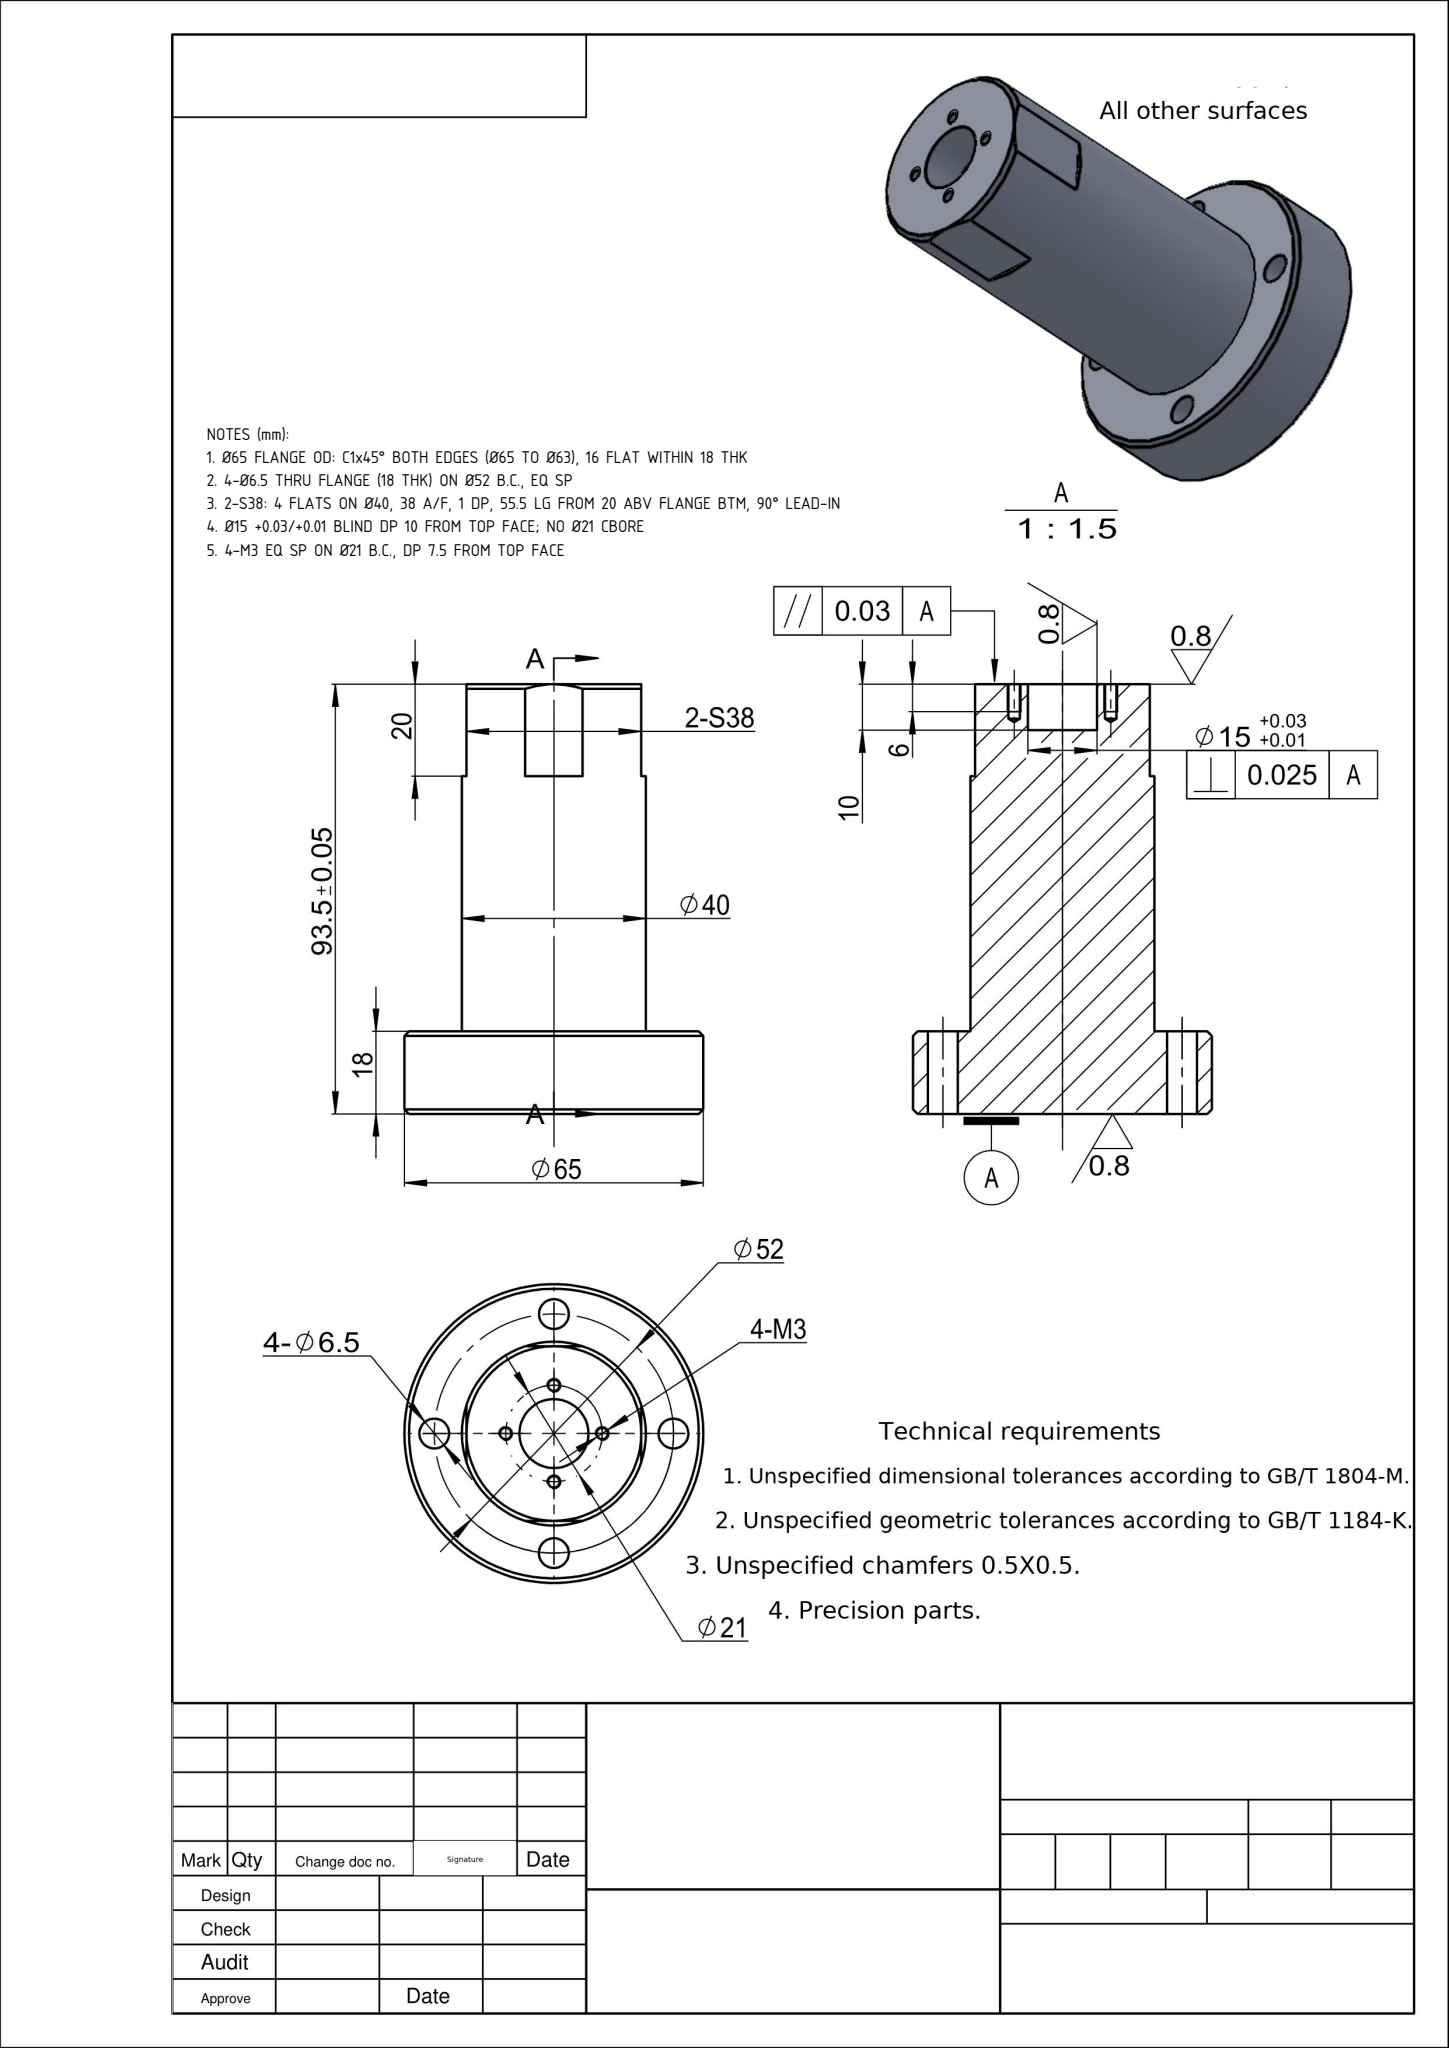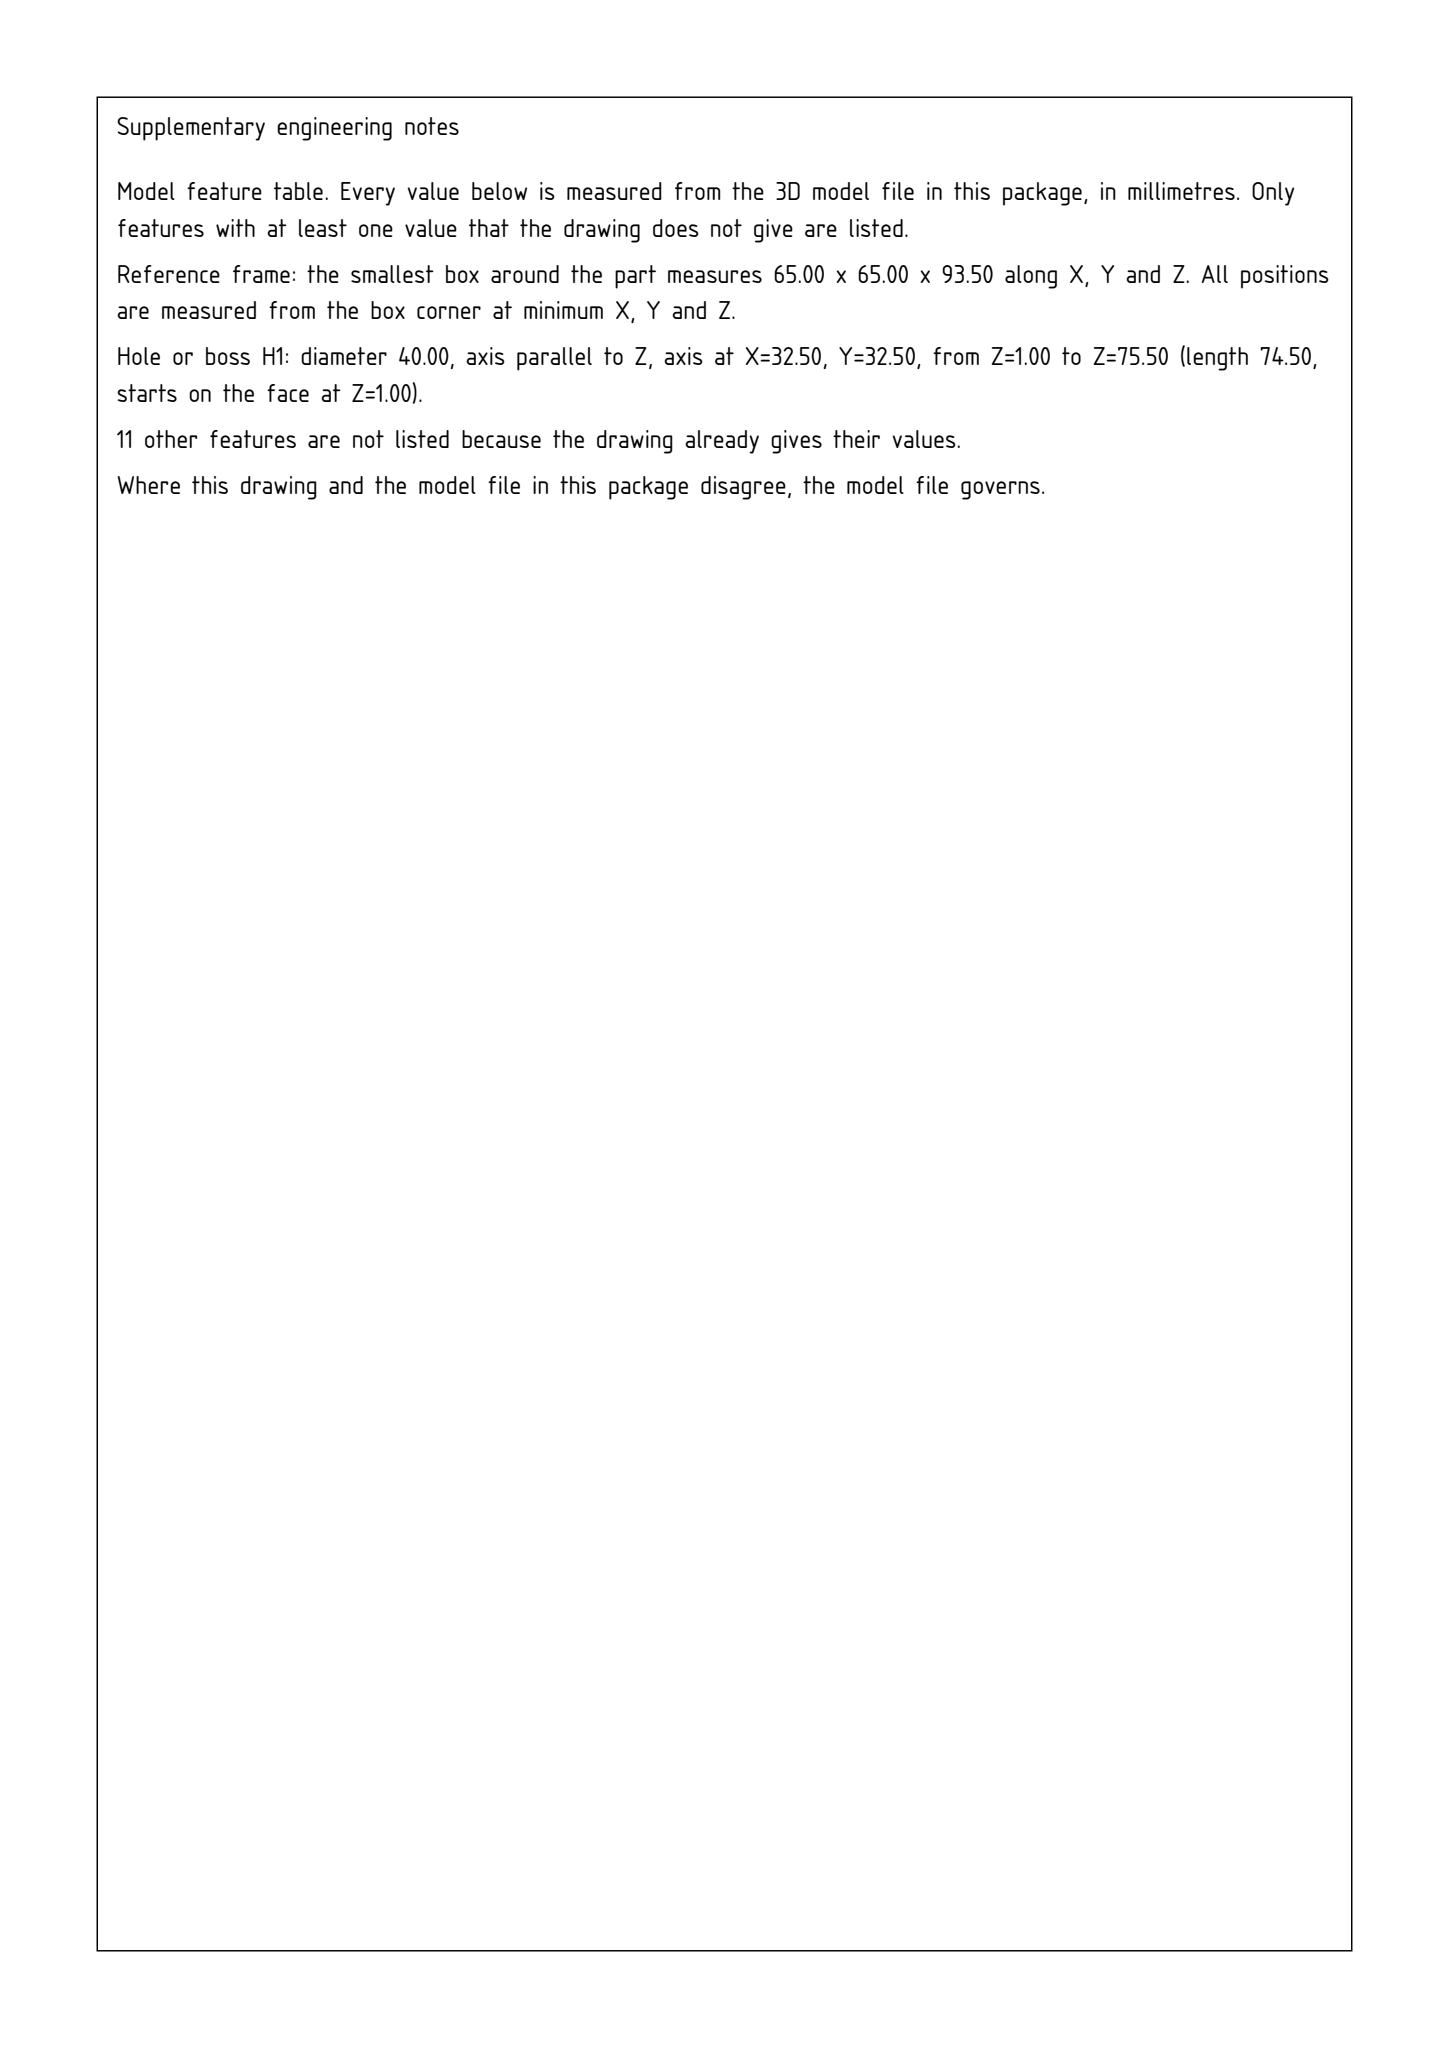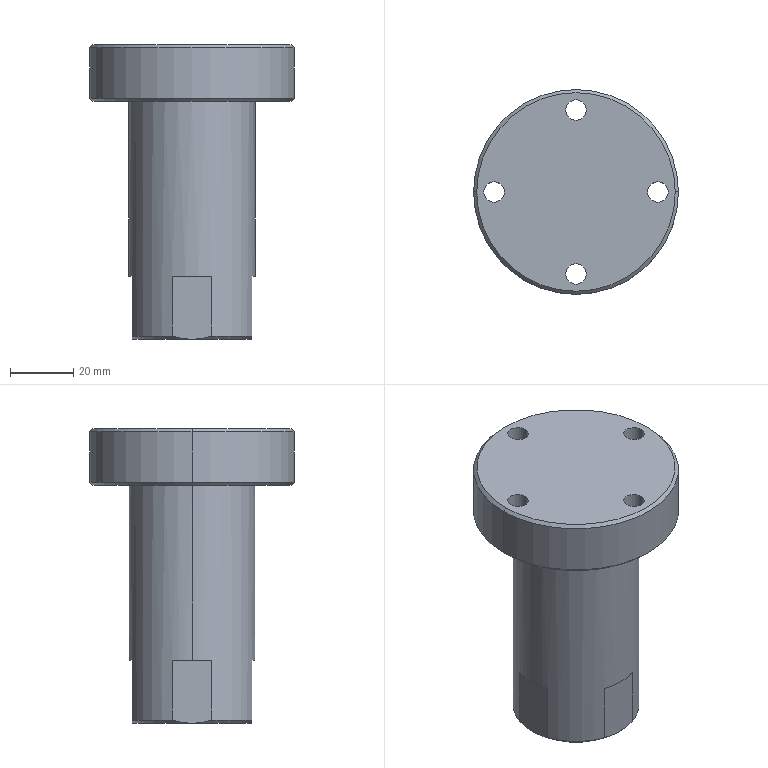Part | SolidWorks | mm | 1 solid | 50 faces | box 65 x 65 x 93.5 mm | volume 149384 mm3 | cylinder 22 | cone 16 | plane 12 | commonest cylinder face diameters 6.5 x8 2.5 x8 15 x2 65 x2 40 x2
Drawing notes:
Ø65 FLANGE OD: C1x45° BOTH EDGES (Ø65 TO Ø63), 16 FLAT WITHIN 18 THK | from the solid: cones [90°,65.0]x2 & [90°,63.0]x2 at both ends of Ø65 cyl len 16, flange 18
4-Ø6.5 THRU FLANGE (18 THK) ON Ø52 B.C., EQ SP | from the solid: 4x cyl Ø6.5 at R26 from axis (6.5/58.5 offsets), length 18 = flange thickness
2-S38: 4 FLATS ON Ø40, 38 A/F, 1 DP, 55.5 LG FROM 20 ABV FLANGE BTM, 90° LEAD-IN | from the solid: planes x=13.5/51.5, y=13.5/51.5 (±19 from CL 32.5); z-planes 20 & 75.5; cones 90° ref Ø38 x4
Ø15 +0.03/+0.01 BLIND DP 10 FROM TOP FACE; NO Ø21 CBORE | from the solid: cyl Ø15 z-axis at (32.5,32.5) len 10 from top z=93.5; no Ø21 cylinder in model
4-M3 EQ SP ON Ø21 B.C., DP 7.5 FROM TOP FACE | from the solid: 4x cyl Ø2.5 at (22,32.5),(32.5,22),(32.5,43),(43,32.5) = R10.5, len 7.5, 118° point
build123d program:
from build123d import *

# Parameters (mm, degrees)
SKETCH1_R           = 32.5
BOSS_EXTRUDE1_DEPTH = 18
SKETCH2_R           = 17.5
BOSS_EXTRUDE2_DEPTH = 5
CHAMFER1_SIZE       = 1
SKETCH3_R           = 20
BOSS_EXTRUDE3_DEPTH = 75.5
SKETCH4_R           = 7.5
CUT_EXTRUDE1_DEPTH  = 10
CIRPATTERN1_COUNT   = 4
CHAMFER2_SIZE       = 1
SKETCH9_OUTSIDE_W   = 93.946
SKETCH9_OUTSIDE_H   = 93.946
SKETCH9_OUTSIDE_W_2 = 38
SKETCH9_OUTSIDE_H_2 = 38
CUT_EXTRUDE3_DEPTH  = 20
CHAMFER3_SIZE       = 1
SKETCH10_W          = 42.613
SKETCH10_H          = 15.277
CUT_EXTRUDE4_DEPTH  = 25
SKETCH11_R          = 3.25
CUT_EXTRUDE5_DEPTH  = 89.39
CIRPATTERN2_COUNT   = 4


with BuildPart() as part:
    # Sketch1 → Boss-Extrude1 (new body)
    with BuildSketch(Plane.XY):
        Circle(SKETCH1_R)
    extrude(amount=BOSS_EXTRUDE1_DEPTH)

    # Sketch2 → Boss-Extrude2 (add)
    with BuildSketch(Plane.XY.offset(18)):
        Circle(SKETCH2_R)
    extrude(amount=BOSS_EXTRUDE2_DEPTH)

    # Chamfer1
    chamfer1_edges = [part.edges().sort_by_distance(p)[0] for p in [
        (-17.5, 0, 23),
    ]]
    chamfer(chamfer1_edges, length=CHAMFER1_SIZE)

    # Sketch3 → Boss-Extrude3 (add)
    with BuildSketch(Plane(origin=(0, 0, 0), x_dir=(-1, 0, 0), z_dir=(0, 0, -1))):
        with Locations(Location((0, 0, 0), (0, 0, 180))):
            Circle(SKETCH3_R)
    extrude(amount=BOSS_EXTRUDE3_DEPTH)

    # Sketch4 → Cut-Extrude1 (cut)
    with BuildSketch(Plane(origin=(0, 0, -75.5), x_dir=(-1, 0, 0), z_dir=(0, 0, -1))):
        Circle(SKETCH4_R)
    extrude(amount=-CUT_EXTRUDE1_DEPTH, mode=Mode.SUBTRACT)

    # Sketch7 → M3 Tapped Hole1 (revolve, cut)
    with BuildSketch(Plane(origin=(-0.00001, -10.5, -75.5), x_dir=(0, 1, 0), z_dir=(1, 0, 0))):
        Polygon((0, 0), (0, 8.251), (1.25, 7.5), (1.25, 0), align=None)
    m3_tapped_hole1 = revolve(axis=Axis((-0.00001, -10.5, -81.85), (0, 0, 1)), mode=Mode.SUBTRACT)

    # CirPattern1: M3 Tapped Hole1 ×4 about axis
    cirpattern1_axis = Axis((0, 0, 0), (0, 0, 1))
    for i in range(1, CIRPATTERN1_COUNT):
        add(m3_tapped_hole1.rotate(cirpattern1_axis, i * 360 / CIRPATTERN1_COUNT), mode=Mode.SUBTRACT)

    # Chamfer2
    chamfer2_edges = [part.edges().sort_by_distance(p)[0] for p in [
        (-20, 0, -75.5),
    ]]
    chamfer(chamfer2_edges, length=CHAMFER2_SIZE)

    # Sketch9 outside → Cut-Extrude3 (cut)
    with BuildSketch(Plane(origin=(0, 0, -75.5), x_dir=(-1, 0, 0), z_dir=(0, 0, -1))):
        Rectangle(SKETCH9_OUTSIDE_W, SKETCH9_OUTSIDE_H)
        Rectangle(SKETCH9_OUTSIDE_W_2, SKETCH9_OUTSIDE_H_2, mode=Mode.SUBTRACT)
    extrude(amount=-CUT_EXTRUDE3_DEPTH, mode=Mode.SUBTRACT)

    # Chamfer3
    chamfer3_edges = [part.edges().sort_by_distance(p)[0] for p in [
        (-32.5, 0, 0),
        (-32.5, 0, 18),
    ]]
    chamfer(chamfer3_edges, length=CHAMFER3_SIZE)

    # Sketch10 → Cut-Extrude4 (cut, symmetric)
    with BuildSketch(Plane(origin=(0, 0, 0), x_dir=(1, 0, 0), z_dir=(0, 1, 0))):
        with Locations((1.343, -25.639)):
            Rectangle(SKETCH10_W, SKETCH10_H)
    extrude(amount=CUT_EXTRUDE4_DEPTH, both=True, mode=Mode.SUBTRACT)

    # Sketch11 → Cut-Extrude5 (cut, through all)
    with BuildSketch(Plane(origin=(0, 0, 0), x_dir=(-1, 0, 0), z_dir=(0, 0, -1))):
        with Locations((0, -26)):
            Circle(SKETCH11_R)
    cut_extrude5 = extrude(amount=-CUT_EXTRUDE5_DEPTH, mode=Mode.SUBTRACT)

    # CirPattern2: Cut-Extrude5 ×4 about axis
    cirpattern2_axis = Axis((0, 0, 0), (0, 0, 1))
    for i in range(1, CIRPATTERN2_COUNT):
        add(cut_extrude5.rotate(cirpattern2_axis, i * 360 / CIRPATTERN2_COUNT), mode=Mode.SUBTRACT)


solid = part.part